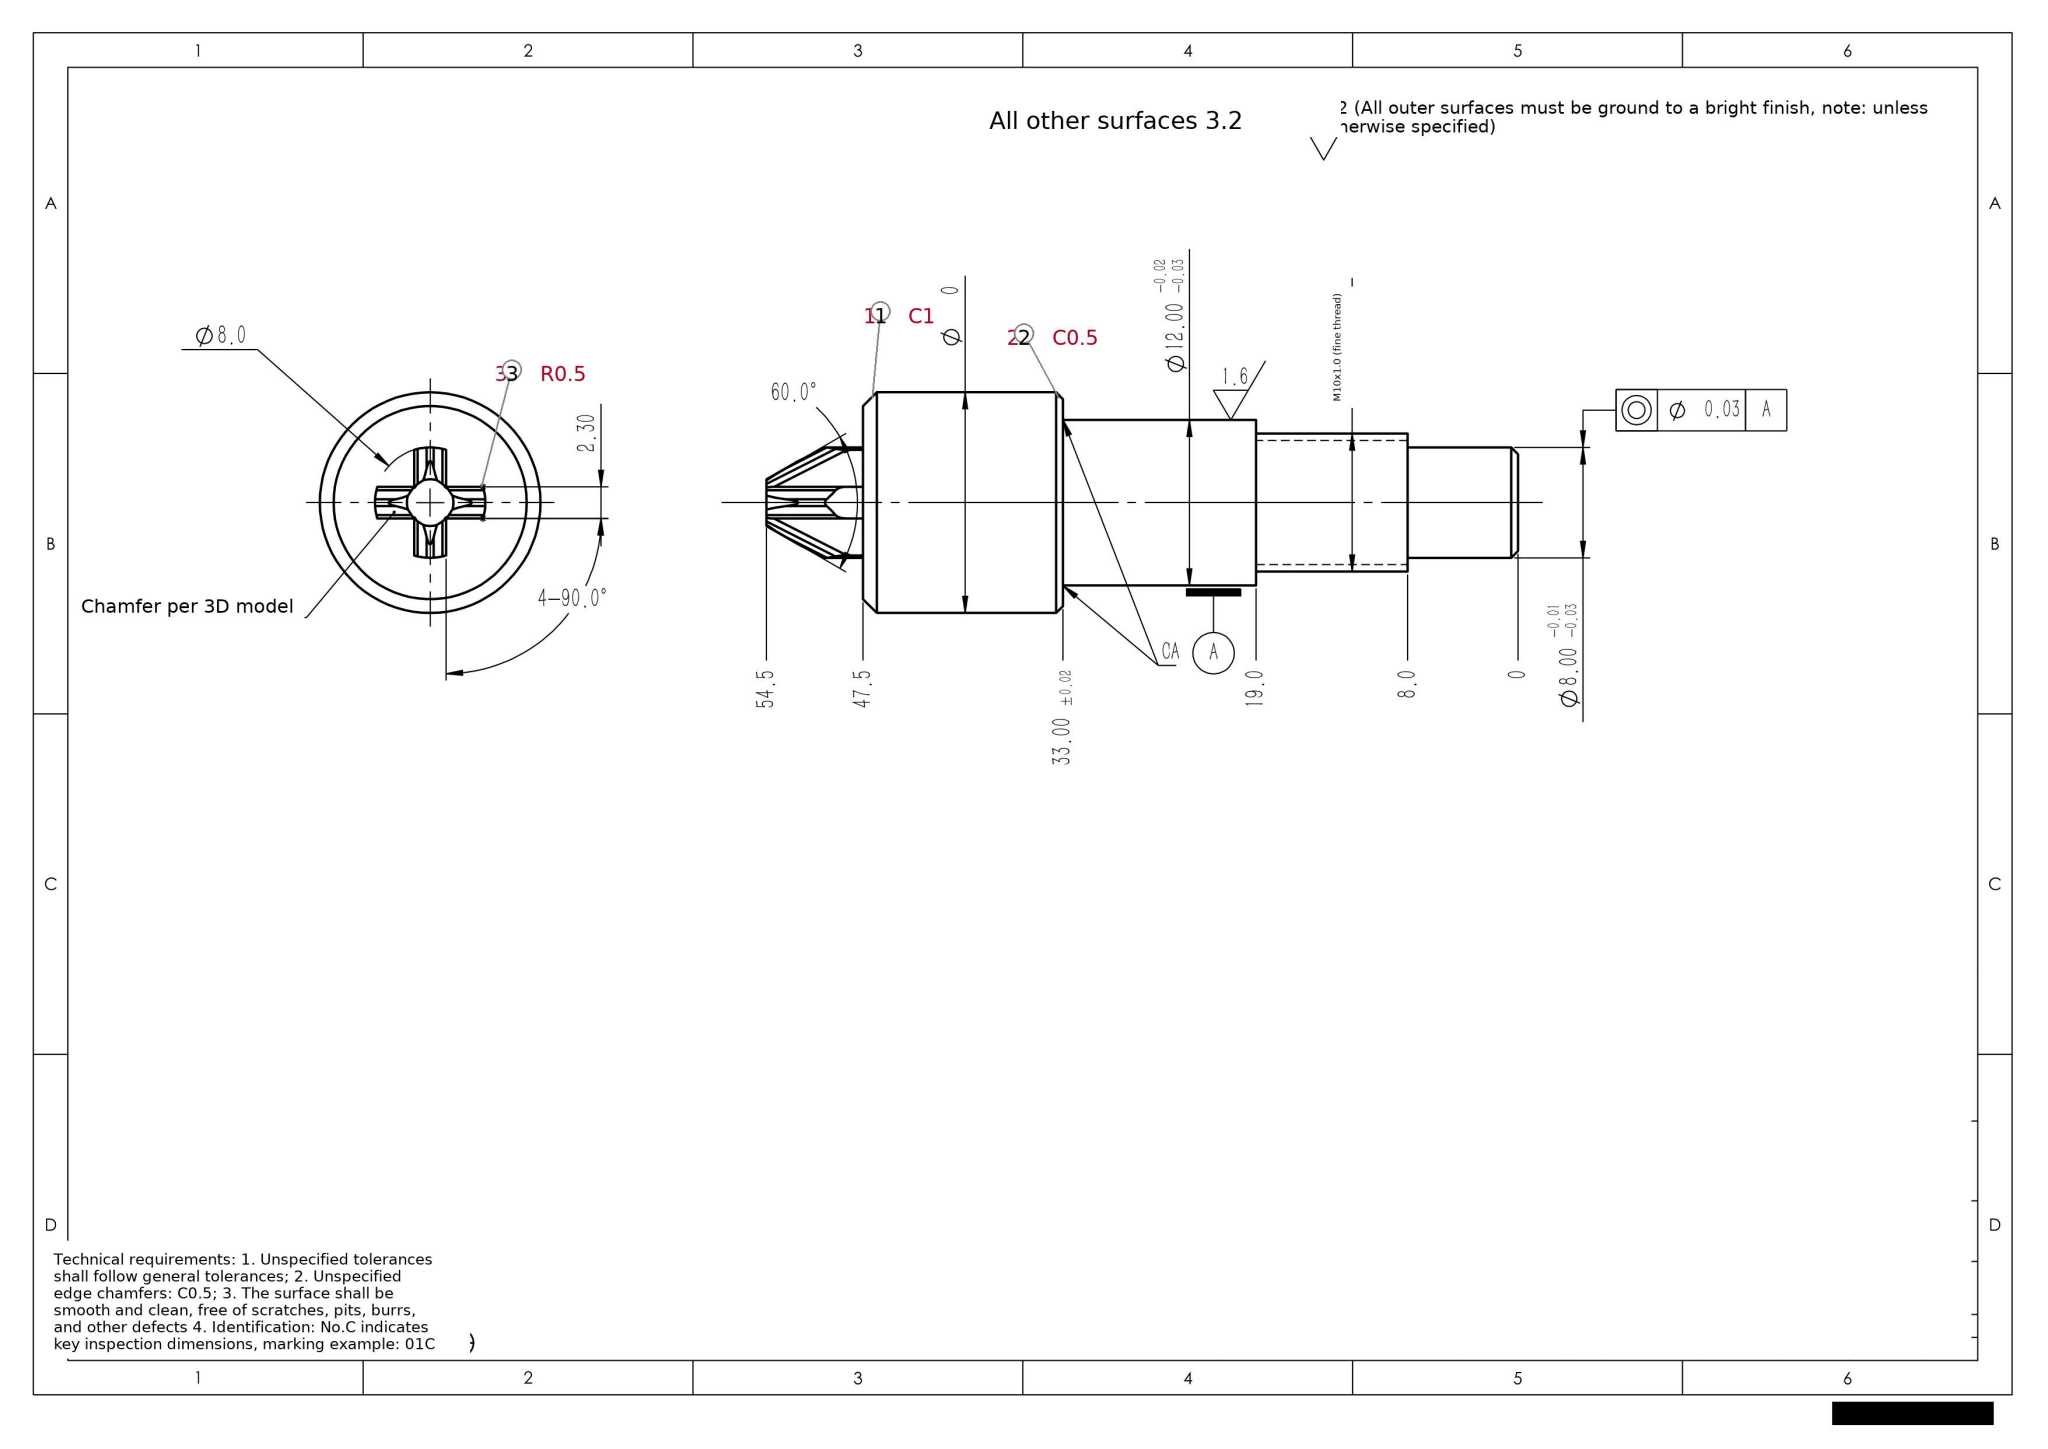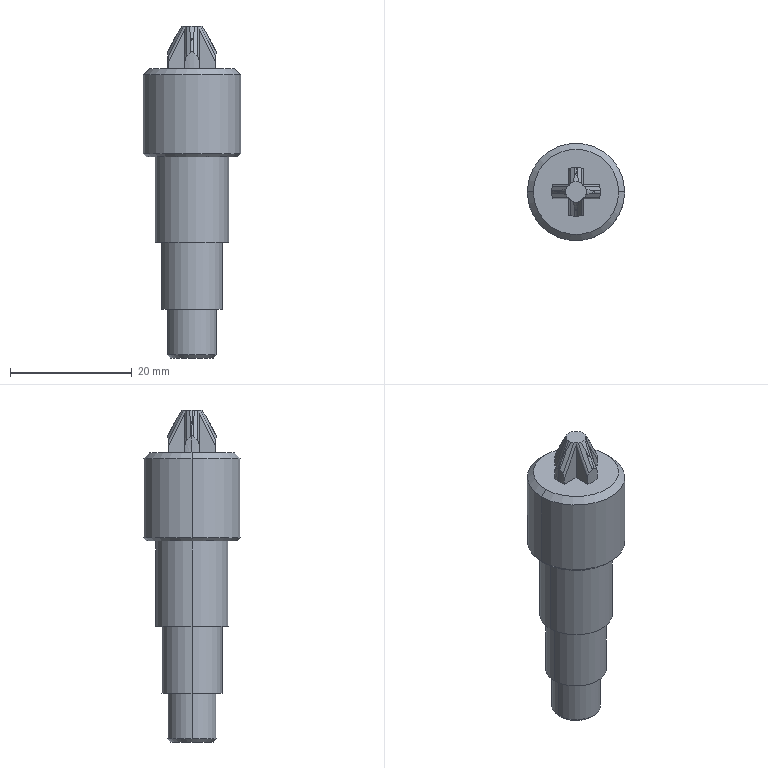Part | SolidWorks | mm | 1 solid | 60 faces | box 16 x 16 x 54.5 mm | volume 5896 mm3 | cylinder 27 | plane 22 | cone 11 | commonest cylinder face diameters 1 x14 8 x7 10 x2 16 x2 12 x2